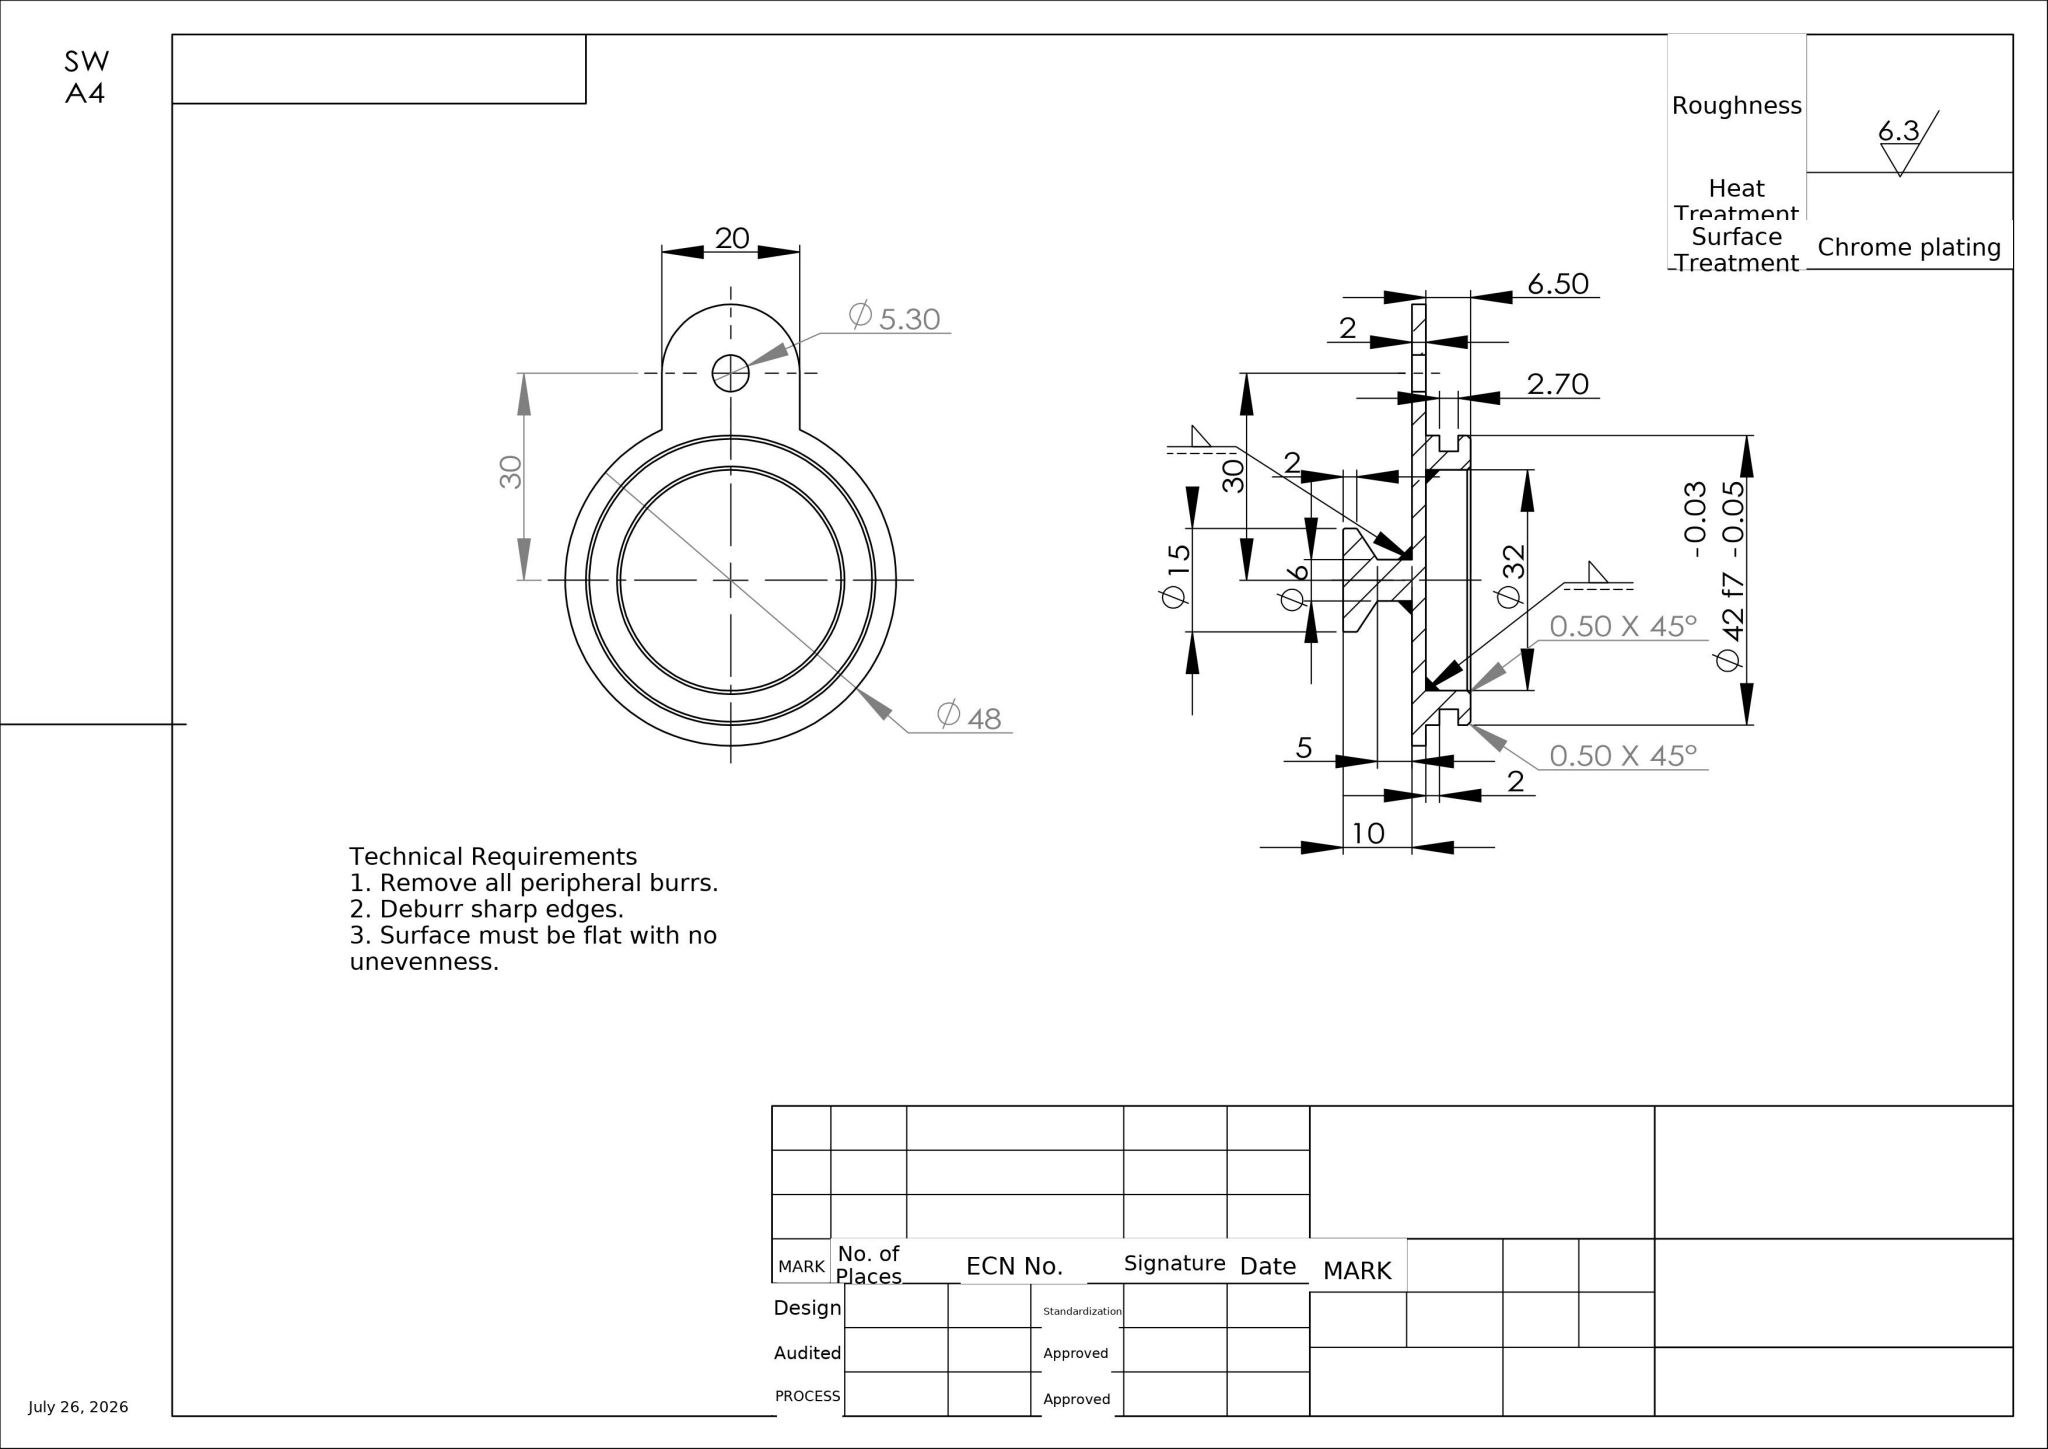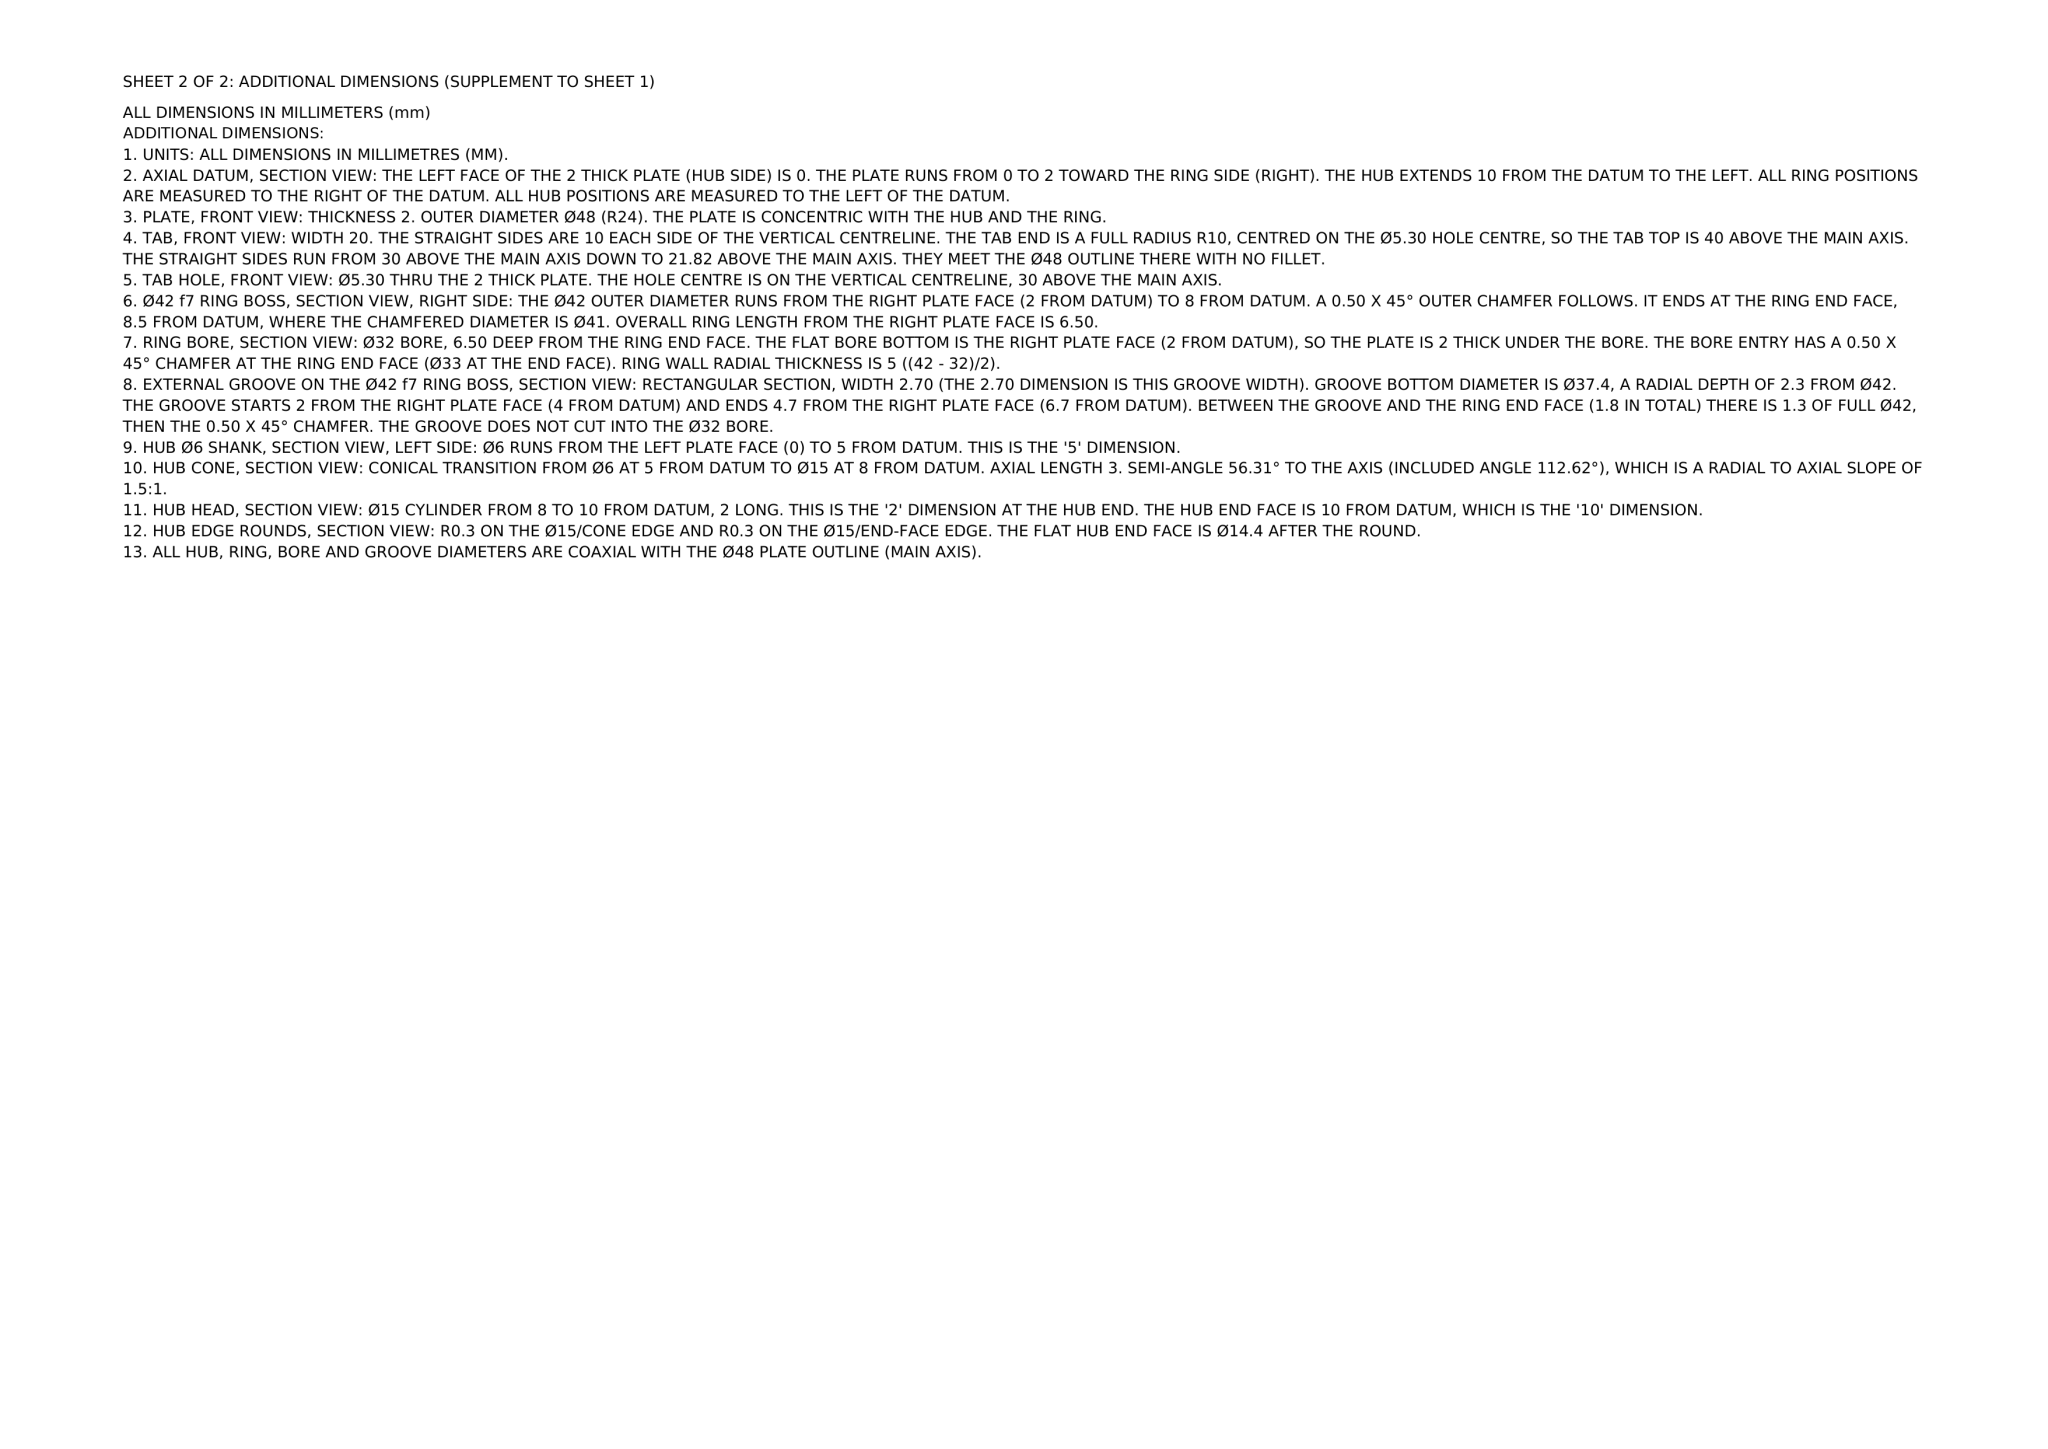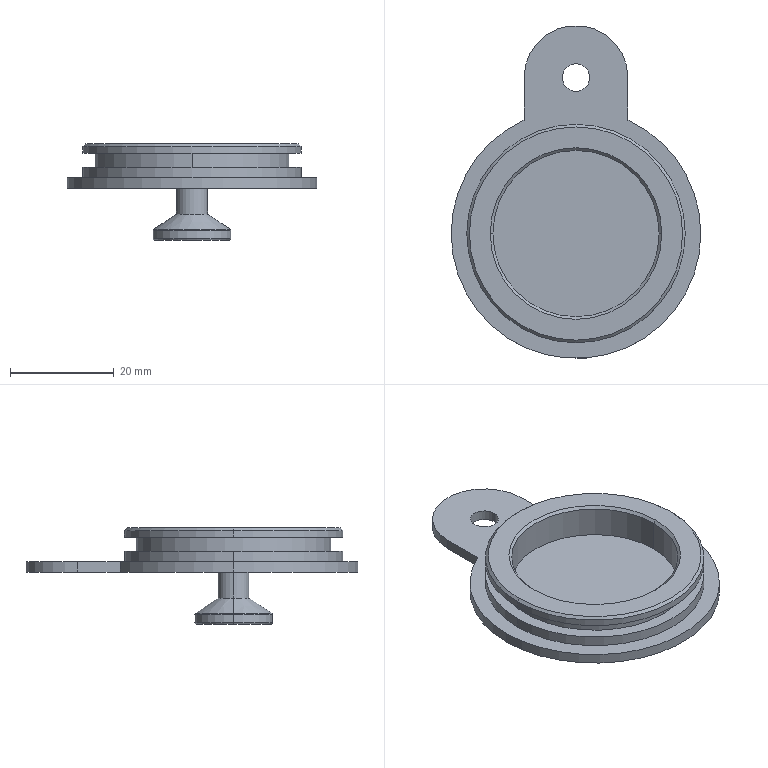Part | NX | mm | 1 solid | 37 faces | box 48 x 64 x 18.5 mm | volume 7901 mm3 | cylinder 18 | plane 9 | cone 6 | torus 4 | commonest cylinder face diameters 42 x4 48 x3 15 x2 6 x2 5.3 x2 37.4 x2 32 x2 20 x1